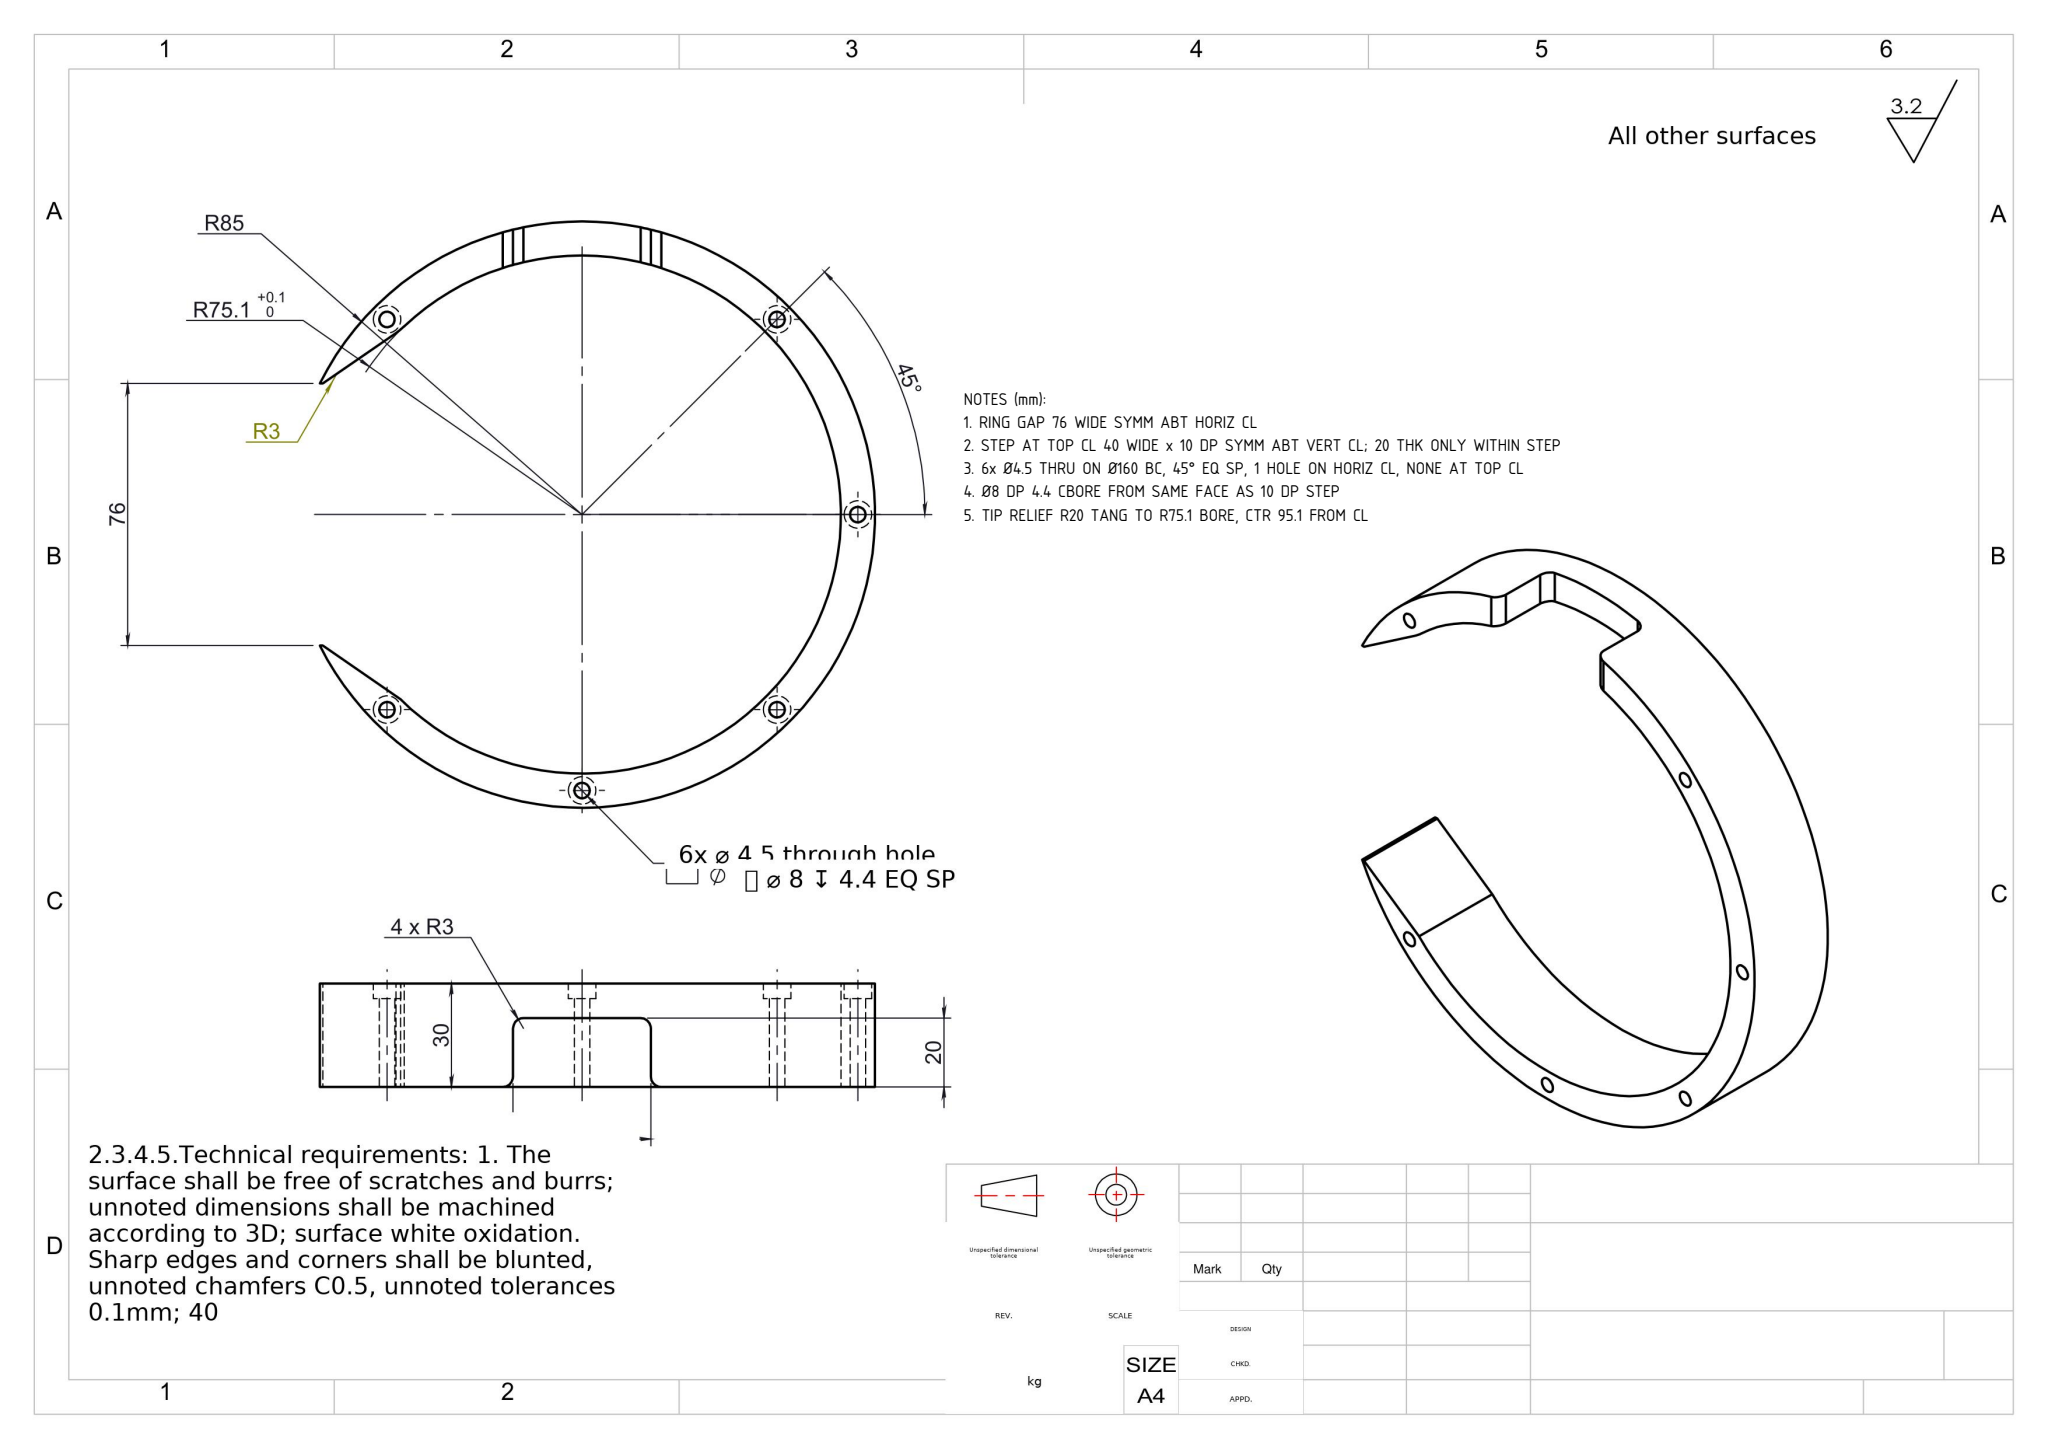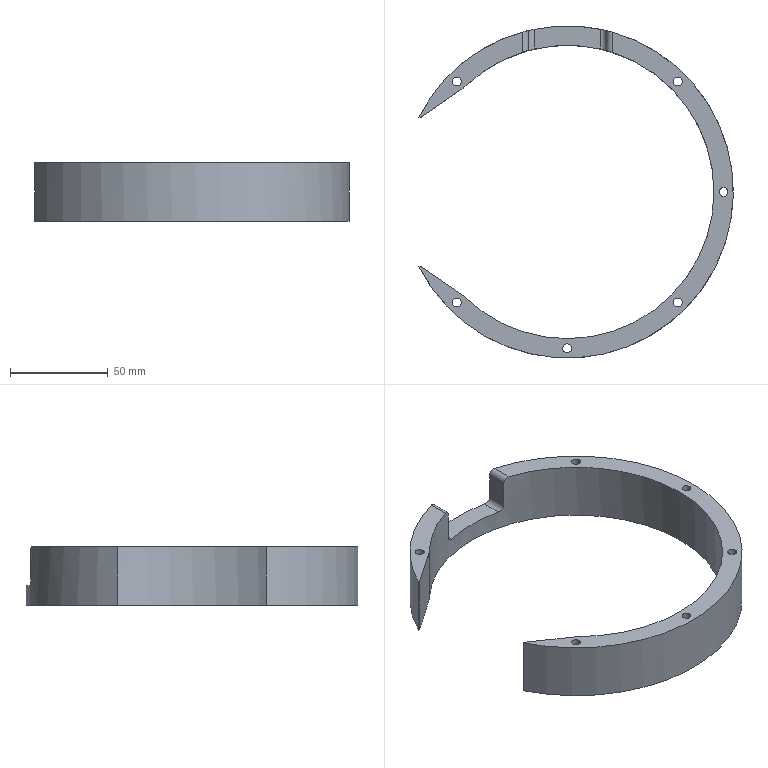Part | SolidWorks | mm | 1 solid | 47 faces | box 161.03 x 170 x 30 mm | volume 109732 mm3 | cylinder 31 | plane 16 | commonest cylinder face diameters 8 x12 4.5 x12 6 x4 170 x1 150.2 x1 40 x1
Drawing notes:
RING GAP 76 WIDE SYMM ABT HORIZ CL | from the solid: End faces y=47 and y=123, ring CL y=85 -> 76 opening, ±38
STEP AT TOP CL 40 WIDE x 10 DP SYMM ABT VERT CL; 20 THK ONLY WITHIN STEP | from the solid: Step walls x=56.03 & 96.03 (40 apart, symm about ring CL x=76.03); floor z=10 in 30 thk body; z=10 floor only between x=56.03 and 96.03
6x Ø4.5 THRU ON Ø160 BC, 45° EQ SP, 1 HOLE ON HORIZ CL, NONE AT TOP CL | from the solid: Ø4.5 holes at (19.46,28.43),(19.46,141.57),(76.03,5),(132.6,28.43),(132.6,141.57),(156.03,85); ring CL (76.03,85) -> R80 = Ø160 BC; angles 0°,±45°,-90°,±135°; gap CL at 180°
Ø8 DP 4.4 CBORE FROM SAME FACE AS 10 DP STEP | from the solid: z=4.4 c'bore floors measured from z=0 face; Ø4.5 thru length 25.6 to z=30; step floor z=10 on same z=0 side
TIP RELIEF R20 TANG TO R75.1 BORE, CTR 95.1 FROM CL | from the solid: Ø40 z-cylinder ctr (10.69,154.09), 95.1 from ring CL = 75.1+20, full 30 length